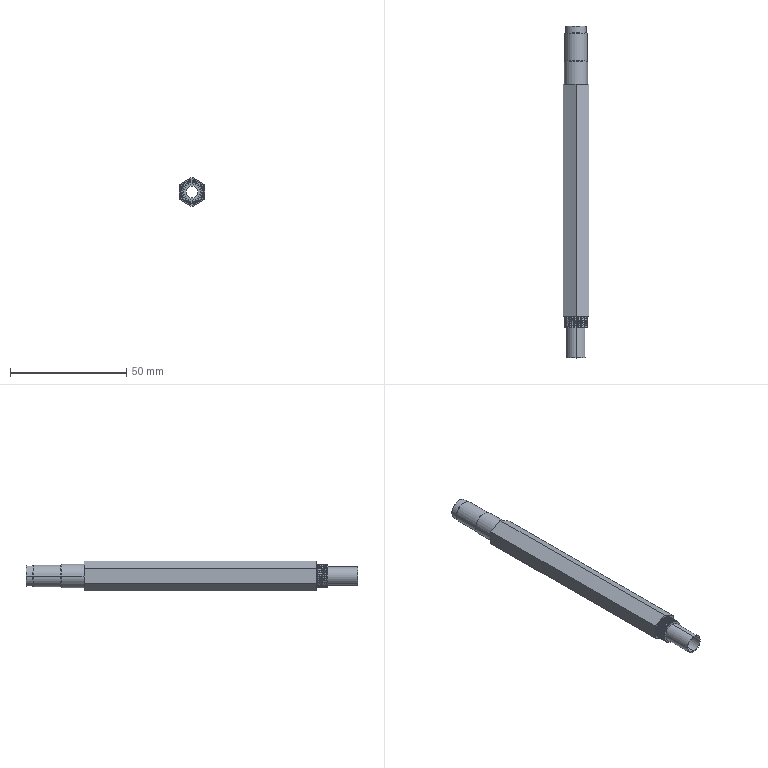Component | SolidWorks | PenBody-1 | 1 solid | 88 faces | volume 2822 mm3 | cylinder 55 | plane 23 | torus 6 | spline 4 | commonest cylinder face diameters 10 x37 9 x6 8 x4 5 x2 8.5 x2 7 x2 9.5 x2